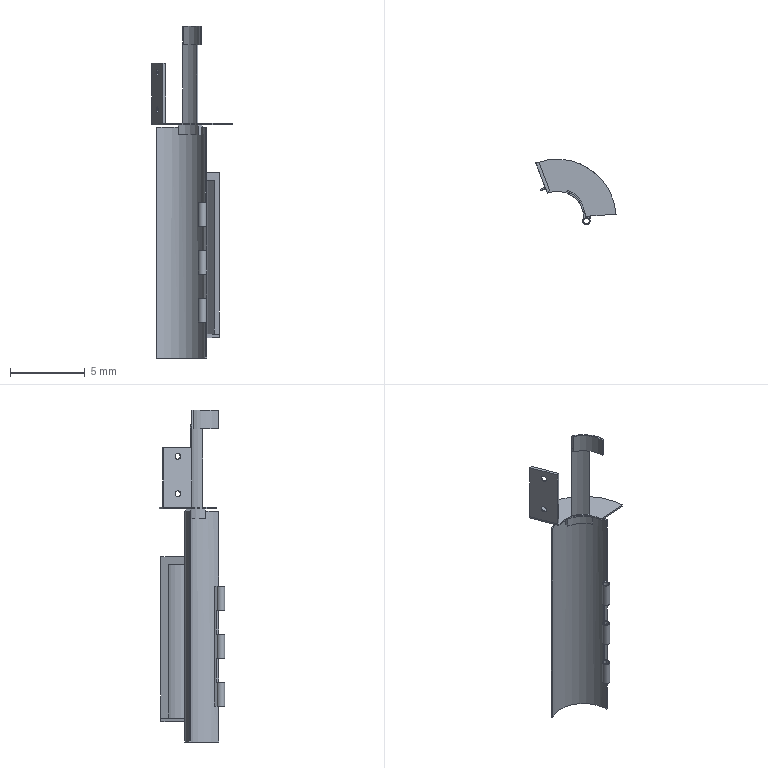Component | NX | HANDLE_SIDE | 3 solids | 69 faces | volume 27 mm3 | plane 46 | cylinder 21 | cone 2 | commonest cylinder face diameters 0.4 x5 0.5 x3 3.8 x3 7.9 x3 4.5 x2 3.6 x2 4.299 x1 6.9 x1